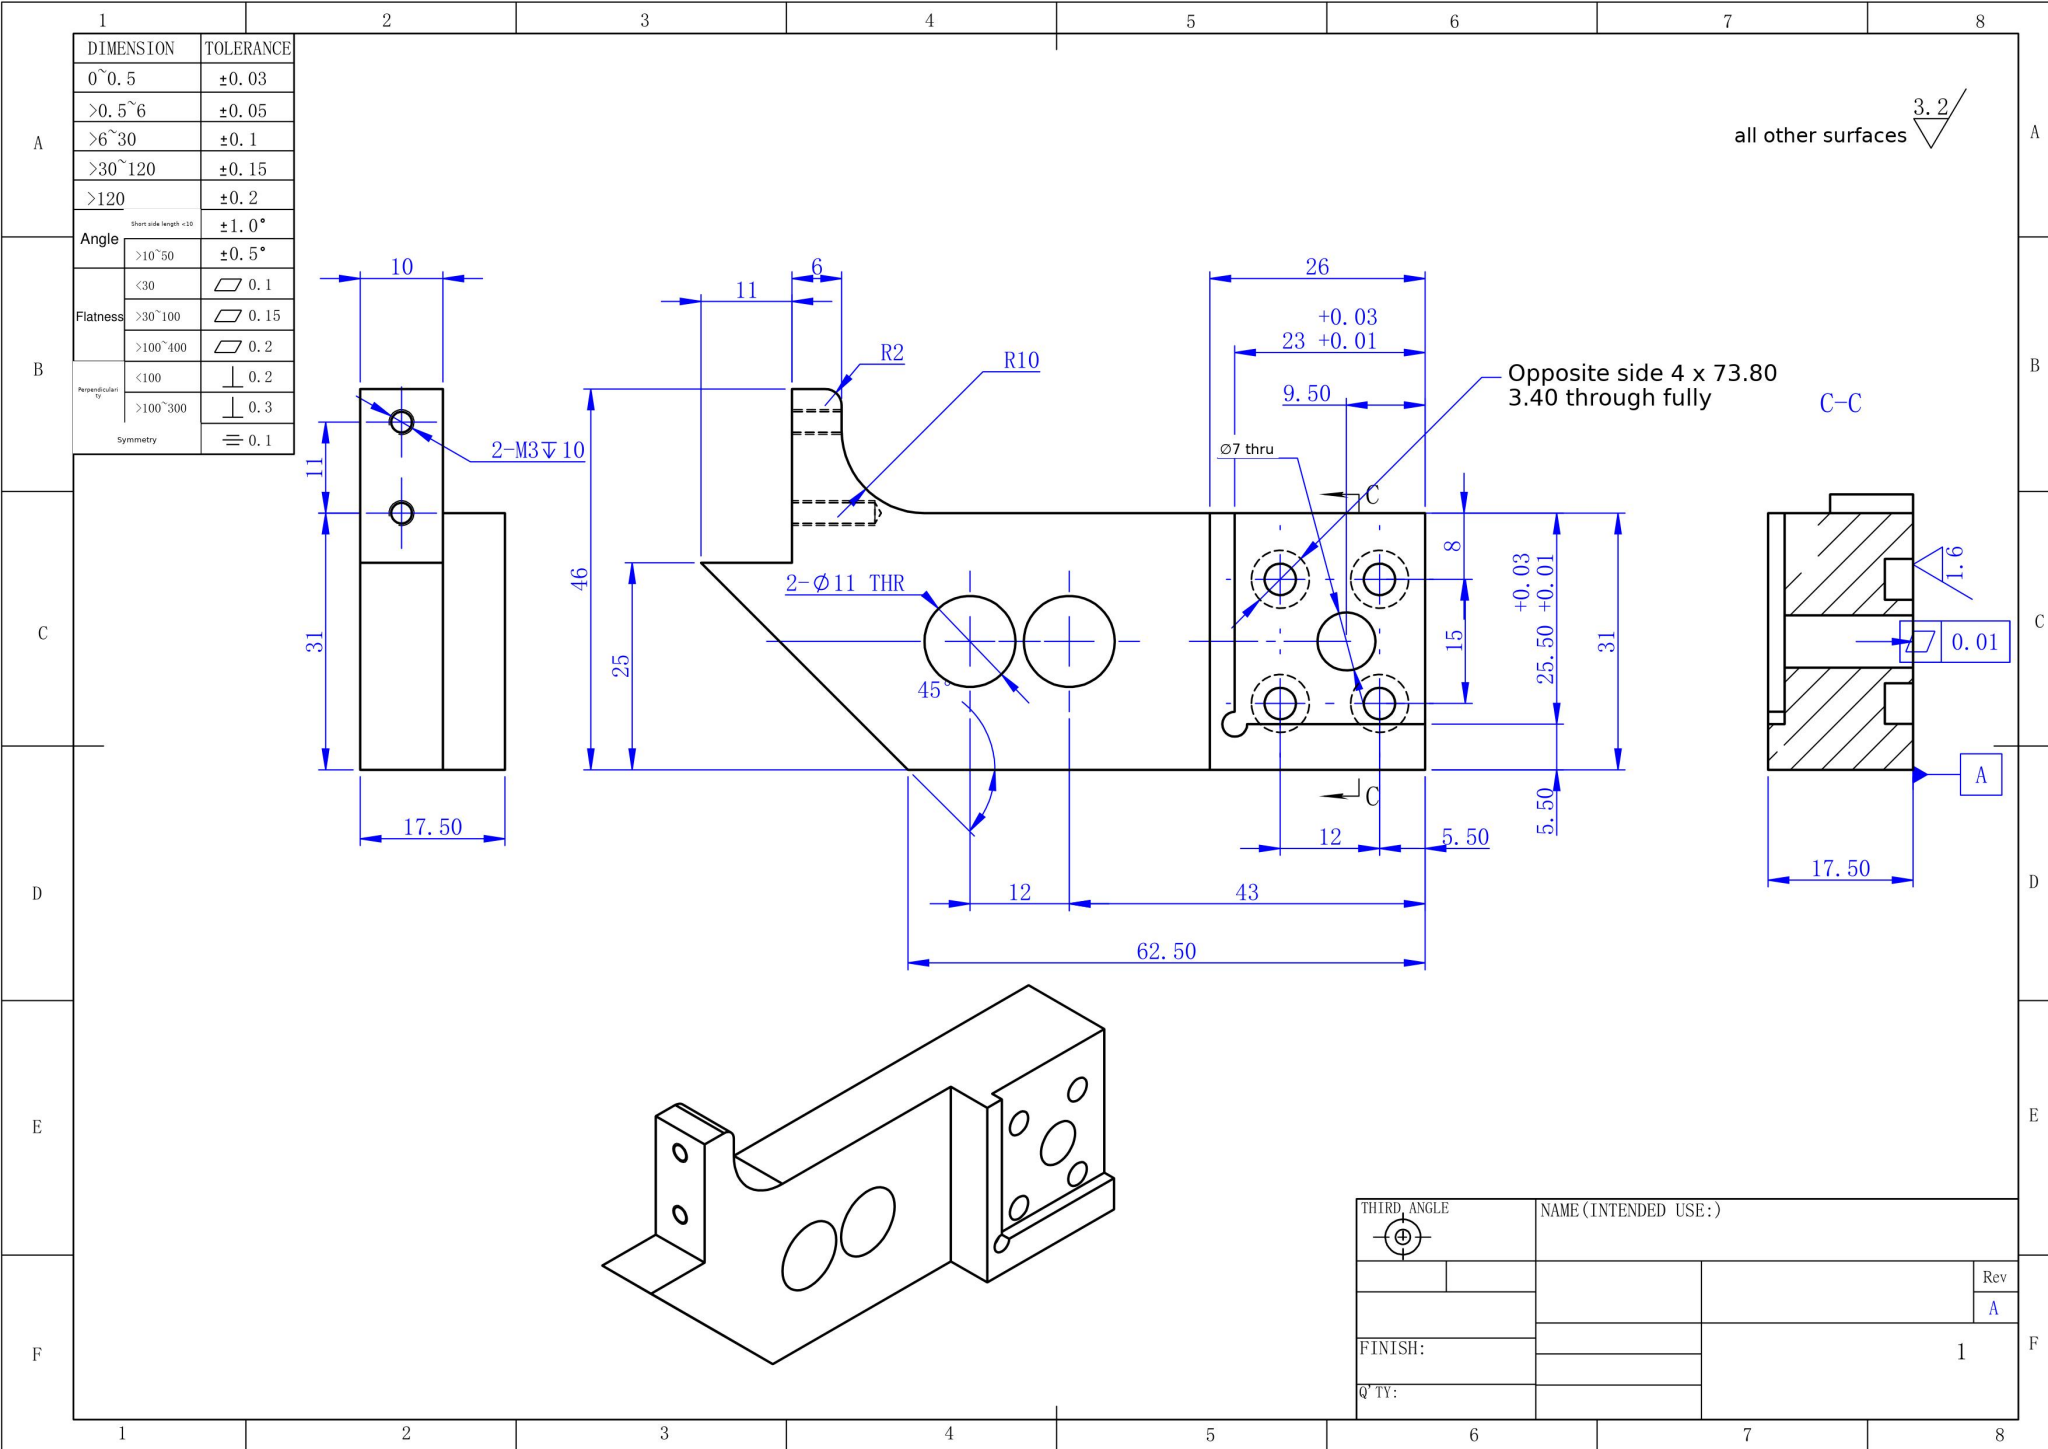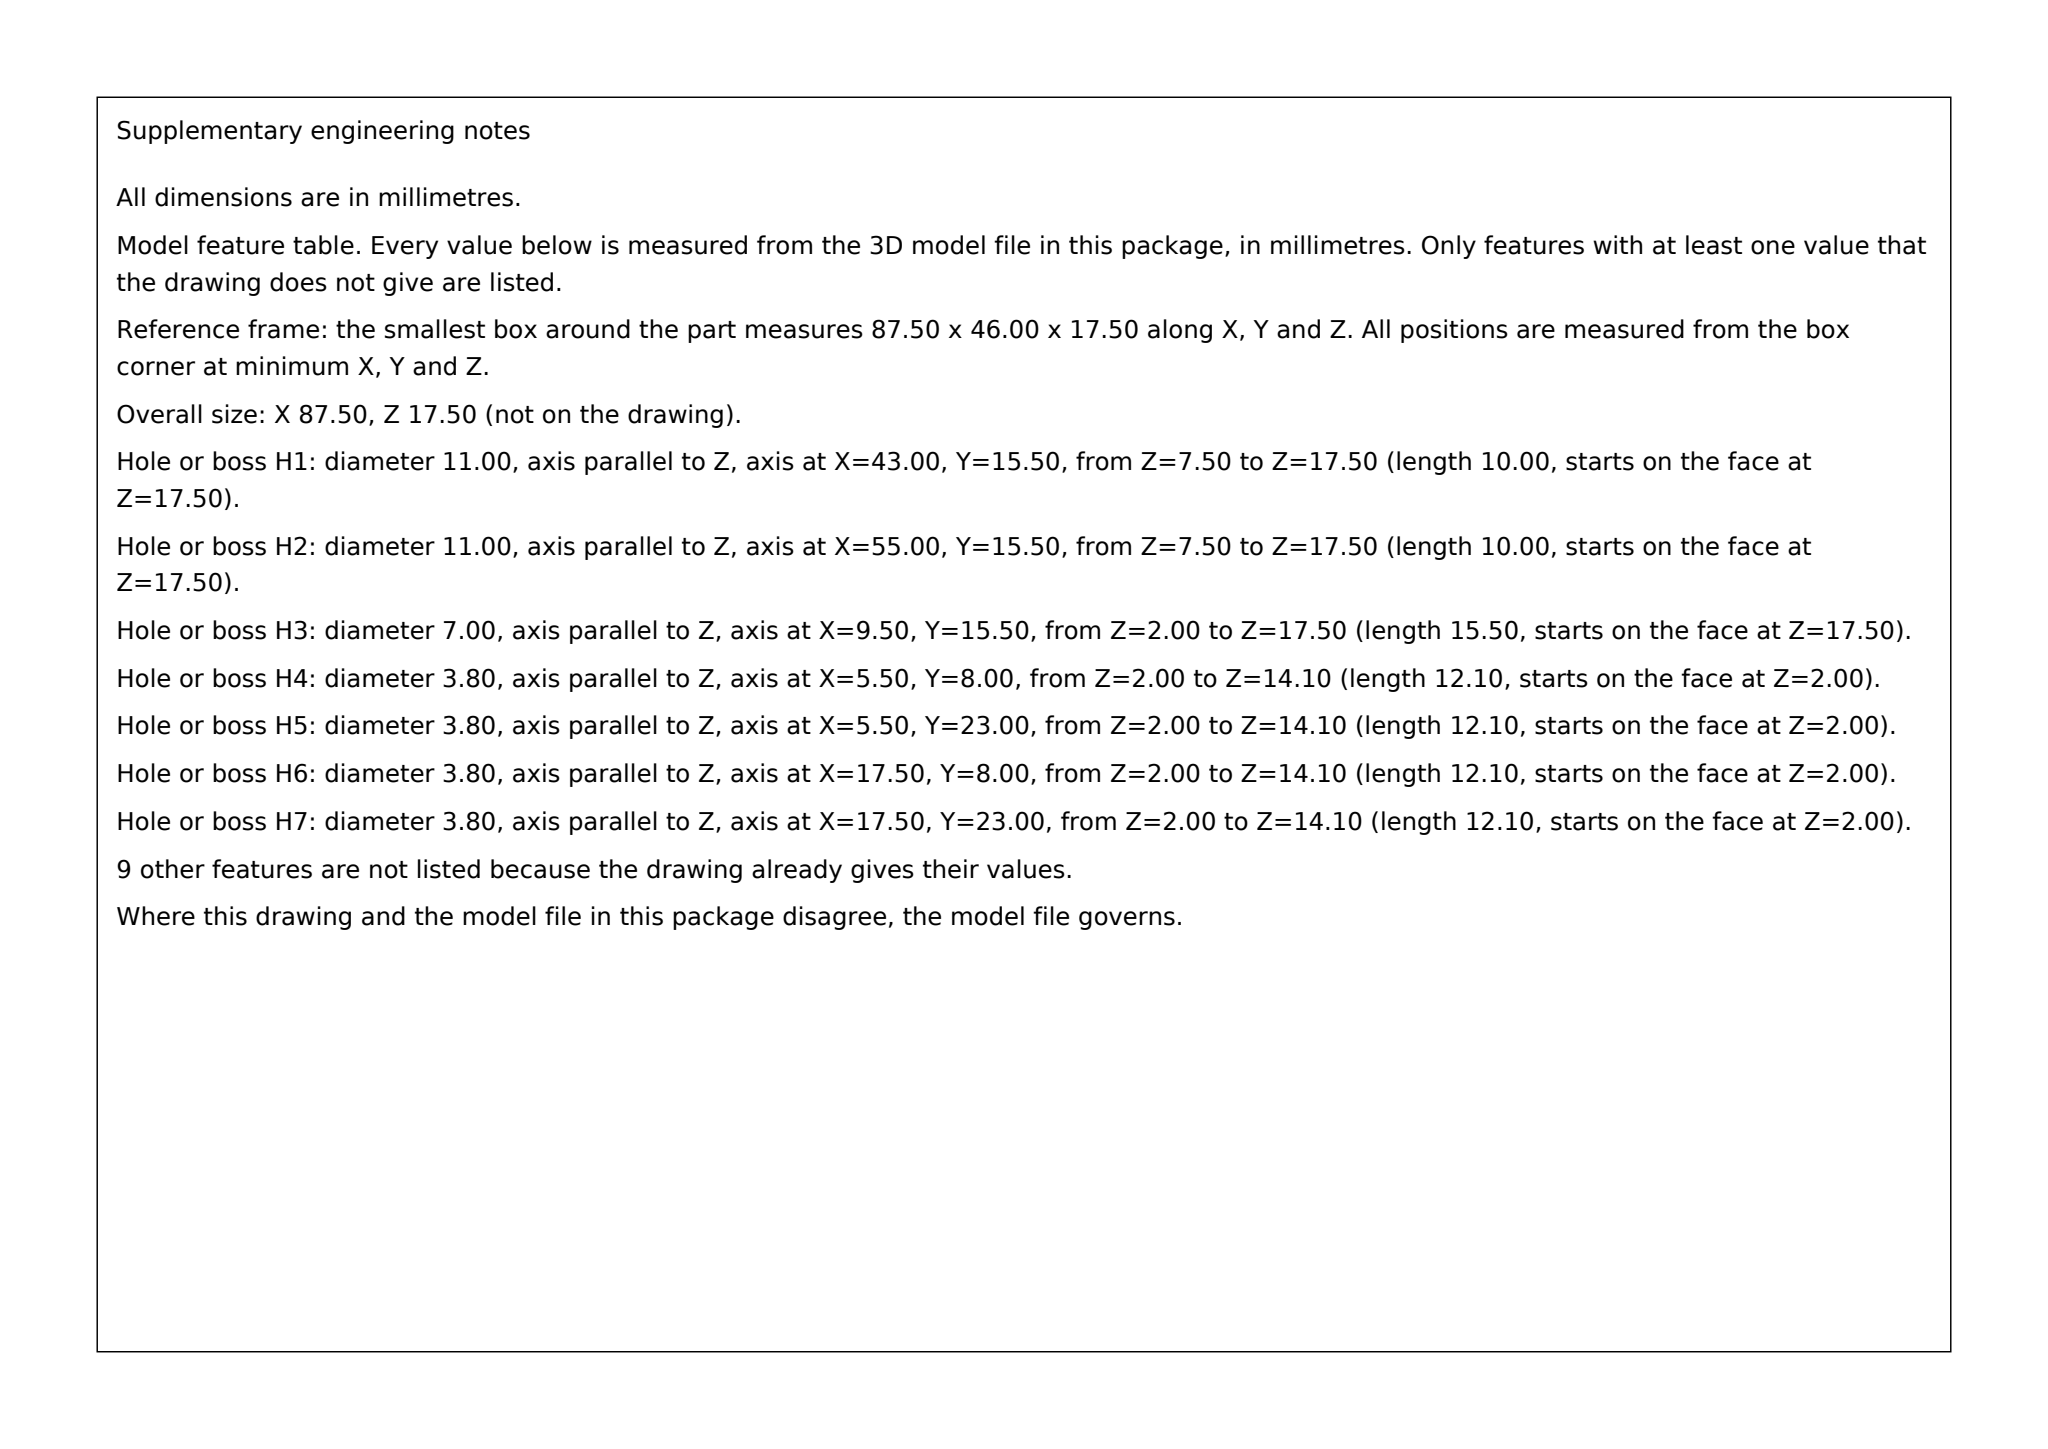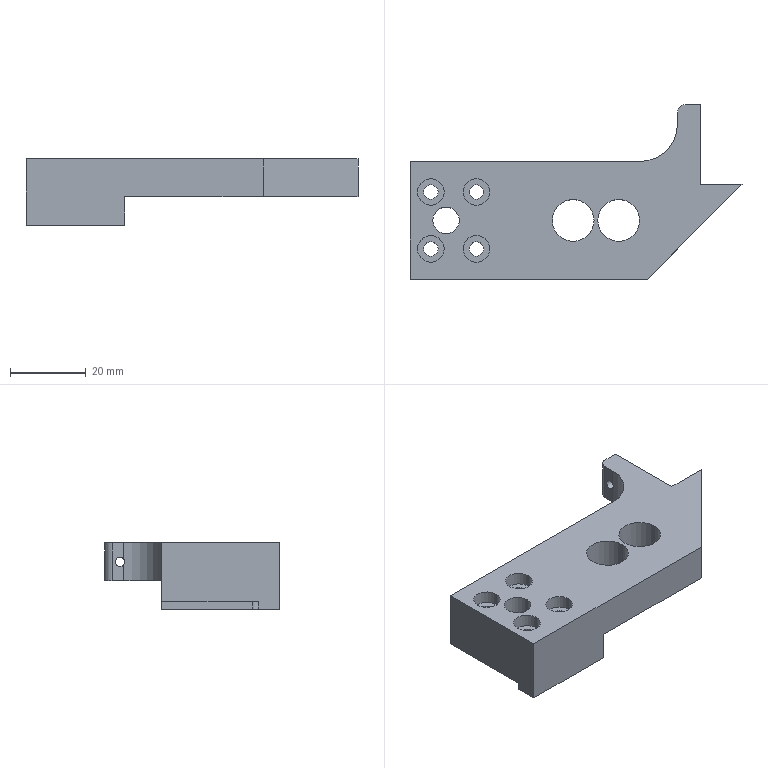Part | SolidWorks | mm | 1 solid | 50 faces | box 87.5 x 46 x 17.5 mm | volume 25658 mm3 | cylinder 29 | plane 19 | cone 2 | commonest cylinder face diameters 7 x10 3.8 x8 2.5 x4 11 x4 20 x1 4 x1 3 x1
build123d program:
from build123d import *

# Parameters (mm, degrees)
BOSS_EXTRUDE1_DEPTH                                  = 17.5
CHAMFER1_SIZE                                        = 25
FILLET1_R                                            = 10
FILLET2_R                                            = 2
SKETCH2_W                                            = 11
SKETCH2_H                                            = 23
CUT_EXTRUDE1_DEPTH                                   = 28.5
SKETCH4_R                                            = 5.5
CUT_EXTRUDE2_DEPTH                                   = 18
M3_TAPPED_HOLE1_D                                    = 2.5
M3_TAPPED_HOLE1_DEPTH                                = 10
M3_TAPPED_HOLE1_TIP                                  = 0.7511
F_7_0_7_DIAMETER_HOLE1_D                             = 7
F_7_0_7_DIAMETER_HOLE1_DEPTH                         = 60
F_7_0_7_DIAMETER_HOLE1_TIP                           = 2.103
HOLE_SIZE_ACCORDING_TO_THE_TYPE_OF_HEXAG_D           = 3.8
HOLE_SIZE_ACCORDING_TO_THE_TYPE_OF_HEXAG_CBORE_D     = 7
HOLE_SIZE_ACCORDING_TO_THE_TYPE_OF_HEXAG_CBORE_DEPTH = 3.4
SKETCH15_W                                           = 23
SKETCH15_H                                           = 25.5
CUT_EXTRUDE4_DEPTH                                   = 2
SKETCH14_R                                           = 1.5
CUT_EXTRUDE3_DEPTH                                   = 2
SKETCH16_W                                           = 63.197
SKETCH16_H                                           = 64.464
CUT_EXTRUDE5_DEPTH                                   = 7.5


with BuildPart() as part:
    # Sketch1 → Boss-Extrude1 (new body)
    with BuildSketch(Plane.XY):
        Polygon((0, 0), (0, 15), (17, 15), (17, -31), (-70.5, -31), (-70.5, 0), align=None)
    extrude(amount=BOSS_EXTRUDE1_DEPTH)

    # Chamfer1
    chamfer1_edges = [part.edges().sort_by_distance(p)[0] for p in [
        (17, -31, 8.75),
    ]]
    chamfer(chamfer1_edges, length=CHAMFER1_SIZE)

    # Fillet1
    fillet1_edges = [part.edges().sort_by_distance(p)[0] for p in [
        (0, 0, 8.75),
    ]]
    fillet(fillet1_edges, radius=FILLET1_R)

    # Fillet2
    fillet2_edges = [part.edges().sort_by_distance(p)[0] for p in [
        (0, 15, 8.75),
    ]]
    fillet(fillet2_edges, radius=FILLET2_R)

    # Sketch2 → Cut-Extrude1 (cut)
    with BuildSketch(Plane.XY.offset(17.5)):
        with Locations((11.5, 5.5)):
            Rectangle(SKETCH2_W, SKETCH2_H)
    extrude(amount=-CUT_EXTRUDE1_DEPTH, mode=Mode.SUBTRACT)

    # Sketch4 → Cut-Extrude2 (cut)
    with BuildSketch(Plane.XY.offset(17.5)):
        with Locations((-27.5, -15.5)):
            Circle(SKETCH4_R)
        with Locations((-15.5, -15.5)):
            Circle(SKETCH4_R)
    extrude(amount=-CUT_EXTRUDE2_DEPTH, mode=Mode.SUBTRACT)

    # M3 Tapped Hole1
    with Locations(Plane(origin=(6, 0, 0), x_dir=(0, 0, -1), z_dir=(1, 0, 0))):
        with Locations((-12.5, 0), (-12.5, 11)):
            Hole(M3_TAPPED_HOLE1_D / 2, depth=M3_TAPPED_HOLE1_DEPTH)
            with Locations((0, 0, -(M3_TAPPED_HOLE1_DEPTH + M3_TAPPED_HOLE1_TIP / 2))):  # 118° drill point
                Cone(0, M3_TAPPED_HOLE1_D / 2, M3_TAPPED_HOLE1_TIP, mode=Mode.SUBTRACT)

    # 7.0 _7_ Diameter Hole1
    with Locations(Plane(origin=(71, 15.5, 17.5), x_dir=(1, 0, 0), z_dir=(0, 0, 1))):
        with Locations((-132, -31)):
            Hole(F_7_0_7_DIAMETER_HOLE1_D / 2, depth=F_7_0_7_DIAMETER_HOLE1_DEPTH)
            with Locations((0, 0, -(F_7_0_7_DIAMETER_HOLE1_DEPTH + F_7_0_7_DIAMETER_HOLE1_TIP / 2))):  # 118° drill point
                Cone(0, F_7_0_7_DIAMETER_HOLE1_D / 2, F_7_0_7_DIAMETER_HOLE1_TIP, mode=Mode.SUBTRACT)

    # Hole size according to the type of hexag (through all)
    with Locations(Plane(origin=(69, 15.5, 17.5), x_dir=(1, 0, 0), z_dir=(0, 0, 1))):
        with Locations((-122, -23.5), (-134, -23.5), (-134, -38.5), (-122, -38.5)):
            CounterBoreHole(HOLE_SIZE_ACCORDING_TO_THE_TYPE_OF_HEXAG_D / 2, HOLE_SIZE_ACCORDING_TO_THE_TYPE_OF_HEXAG_CBORE_D / 2, HOLE_SIZE_ACCORDING_TO_THE_TYPE_OF_HEXAG_CBORE_DEPTH)

    # Sketch15 → Cut-Extrude4 (cut)
    with BuildSketch(Plane(origin=(0, 0, 0), x_dir=(-1, 0, 0), z_dir=(0, 0, -1))):
        with Locations((59, -12.75)):
            Rectangle(SKETCH15_W, SKETCH15_H)
    extrude(amount=-CUT_EXTRUDE4_DEPTH, mode=Mode.SUBTRACT)

    # Sketch14 → Cut-Extrude3 (cut)
    with BuildSketch(Plane(origin=(0, 0, 0), x_dir=(-1, 0, 0), z_dir=(0, 0, -1))):
        with Locations((47.5, -25.5)):
            Circle(SKETCH14_R)
    extrude(amount=-CUT_EXTRUDE3_DEPTH, mode=Mode.SUBTRACT)

    # Sketch16 → Cut-Extrude5 (cut)
    with BuildSketch(Plane(origin=(0, 0, 0), x_dir=(-1, 0, 0), z_dir=(0, 0, -1))):
        with Locations((12.902, -10.535)):
            Rectangle(SKETCH16_W, SKETCH16_H)
    extrude(amount=-CUT_EXTRUDE5_DEPTH, mode=Mode.SUBTRACT)


solid = part.part